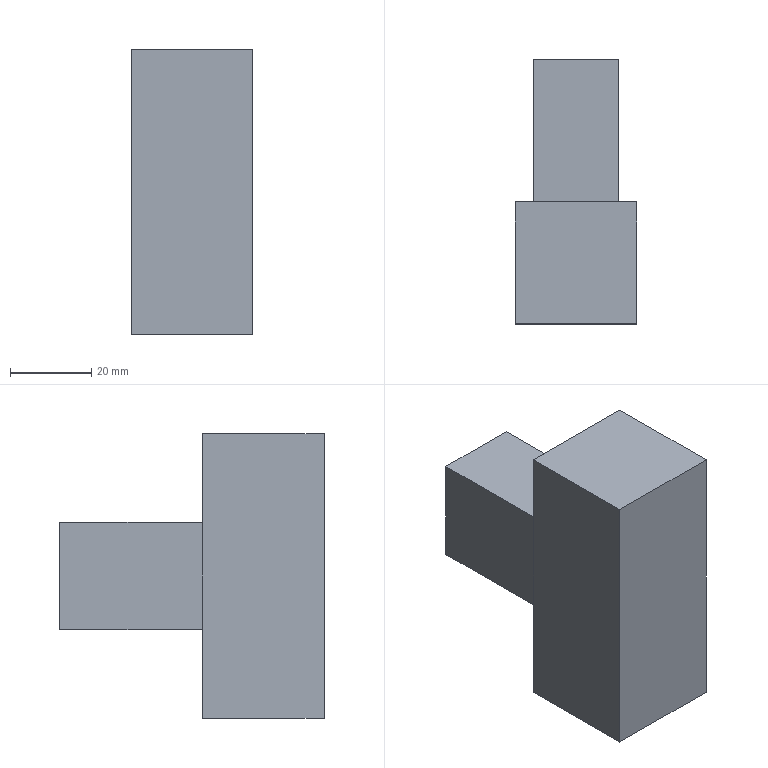Component | SolidWorks | HH54PIntermediateRelay-3 | 1 solid | 11 faces | box 30 x 65 x 70 mm | volume 82478 mm3 | plane 11
STEP:
#1=CARTESIAN_POINT('',(12.461,-0.7598,23.26));
#2=VERTEX_POINT('',#1);
#3=CARTESIAN_POINT('',(12.461,-0.7598,26.016));
#4=VERTEX_POINT('',#3);
#5=CARTESIAN_POINT('',(12.461,-0.7598,23.26));
#6=DIRECTION('',(0.,0.,1.));
#7=VECTOR('',#6,39.37);
#8=LINE('',#5,#7);
#9=EDGE_CURVE('',#2,#4,#8,.T.);
#10=ORIENTED_EDGE('',*,*,#9,.T.);
#11=CARTESIAN_POINT('',(13.643,-0.7598,26.016));
#12=VERTEX_POINT('',#11);
#13=CARTESIAN_POINT('',(12.461,-0.7598,26.016));
#14=DIRECTION('',(1.,0.,0.));
#15=VECTOR('',#14,39.37);
#16=LINE('',#13,#15);
#17=EDGE_CURVE('',#4,#12,#16,.T.);
#18=ORIENTED_EDGE('',*,*,#17,.T.);
#19=CARTESIAN_POINT('',(13.643,-0.7598,23.26));
#20=VERTEX_POINT('',#19);
#21=CARTESIAN_POINT('',(13.643,-0.7598,23.26));
#22=DIRECTION('',(-0.,-0.,-1.));
#23=VECTOR('',#22,39.37);
#24=LINE('',#21,#23);
#25=EDGE_CURVE('',#12,#20,#24,.T.);
#26=ORIENTED_EDGE('',*,*,#25,.T.);
#27=CARTESIAN_POINT('',(12.461,-0.7598,23.26));
#28=DIRECTION('',(-1.,0.,0.));
#29=VECTOR('',#28,39.37);
#30=LINE('',#27,#29);
#31=EDGE_CURVE('',#20,#2,#30,.T.);
#32=ORIENTED_EDGE('',*,*,#31,.T.);
#33=EDGE_LOOP('',(#10,#18,#26,#32));
#34=FACE_OUTER_BOUND('',#33,.T.);
#35=CARTESIAN_POINT('',(12.639,-0.7598,25.16));
#36=VERTEX_POINT('',#35);
#37=CARTESIAN_POINT('',(13.465,-0.7598,25.16));
#38=VERTEX_POINT('',#37);
#39=CARTESIAN_POINT('',(12.639,-0.7598,25.16));
#40=DIRECTION('',(1.,0.,0.));
#41=VECTOR('',#40,39.37);
#42=LINE('',#39,#41);
#43=EDGE_CURVE('',#36,#38,#42,.T.);
#44=ORIENTED_EDGE('',*,*,#43,.F.);
#45=CARTESIAN_POINT('',(12.639,-0.7598,24.116));
#46=VERTEX_POINT('',#45);
#47=CARTESIAN_POINT('',(12.639,-0.7598,24.116));
#48=DIRECTION('',(0.,0.,1.));
#49=VECTOR('',#48,39.37);
#50=LINE('',#47,#49);
#51=EDGE_CURVE('',#46,#36,#50,.T.);
#52=ORIENTED_EDGE('',*,*,#51,.F.);
#53=CARTESIAN_POINT('',(13.465,-0.7598,24.116));
#54=VERTEX_POINT('',#53);
#55=CARTESIAN_POINT('',(12.639,-0.7598,24.116));
#56=DIRECTION('',(-1.,0.,0.));
#57=VECTOR('',#56,39.37);
#58=LINE('',#55,#57);
#59=EDGE_CURVE('',#54,#46,#58,.T.);
#60=ORIENTED_EDGE('',*,*,#59,.F.);
#61=CARTESIAN_POINT('',(13.465,-0.7598,24.116));
#62=DIRECTION('',(-0.,-0.,-1.));
#63=VECTOR('',#62,39.37);
#64=LINE('',#61,#63);
#65=EDGE_CURVE('',#38,#54,#64,.T.);
#66=ORIENTED_EDGE('',*,*,#65,.F.);
#67=EDGE_LOOP('',(#44,#52,#60,#66));
#68=FACE_BOUND('',#67,.T.);
#69=CARTESIAN_POINT('',(13.267,-0.7598,24.309));
#70=DIRECTION('',(0.,1.,-0.));
#71=DIRECTION('',(1.,0.,0.));
#72=AXIS2_PLACEMENT_3D('',#69,#70,#71);
#73=PLANE('',#72);
#74=ADVANCED_FACE('',(#34,#68),#73,.T.);
#75=CARTESIAN_POINT('',(12.461,-1.941,23.26));
#76=VERTEX_POINT('',#75);
#77=CARTESIAN_POINT('',(12.461,-1.941,26.016));
#78=VERTEX_POINT('',#77);
#79=CARTESIAN_POINT('',(12.461,-1.941,23.26));
#80=DIRECTION('',(0.,0.,1.));
#81=VECTOR('',#80,39.37);
#82=LINE('',#79,#81);
#83=EDGE_CURVE('',#76,#78,#82,.T.);
#84=ORIENTED_EDGE('',*,*,#83,.T.);
#85=CARTESIAN_POINT('',(12.461,-0.7598,26.016));
#86=DIRECTION('',(0.,-1.,0.));
#87=VECTOR('',#86,39.37);
#88=LINE('',#85,#87);
#89=EDGE_CURVE('',#4,#78,#88,.T.);
#90=ORIENTED_EDGE('',*,*,#89,.F.);
#91=ORIENTED_EDGE('',*,*,#9,.F.);
#92=CARTESIAN_POINT('',(12.461,-0.7598,23.26));
#93=DIRECTION('',(0.,-1.,0.));
#94=VECTOR('',#93,39.37);
#95=LINE('',#92,#94);
#96=EDGE_CURVE('',#2,#76,#95,.T.);
#97=ORIENTED_EDGE('',*,*,#96,.T.);
#98=EDGE_LOOP('',(#84,#90,#91,#97));
#99=FACE_OUTER_BOUND('',#98,.T.);
#100=CARTESIAN_POINT('',(12.461,-0.7598,23.26));
#101=DIRECTION('',(1.,0.,0.));
#102=DIRECTION('',(0.,-1.,0.));
#103=AXIS2_PLACEMENT_3D('',#100,#101,#102);
#104=PLANE('',#103);
#105=ADVANCED_FACE('',(#99),#104,.F.);
#106=CARTESIAN_POINT('',(13.643,-1.941,26.016));
#107=VERTEX_POINT('',#106);
#108=CARTESIAN_POINT('',(12.461,-1.941,26.016));
#109=DIRECTION('',(1.,0.,0.));
#110=VECTOR('',#109,39.37);
#111=LINE('',#108,#110);
#112=EDGE_CURVE('',#78,#107,#111,.T.);
#113=ORIENTED_EDGE('',*,*,#112,.T.);
#114=CARTESIAN_POINT('',(13.643,-0.7598,26.016));
#115=DIRECTION('',(0.,-1.,0.));
#116=VECTOR('',#115,39.37);
#117=LINE('',#114,#116);
#118=EDGE_CURVE('',#12,#107,#117,.T.);
#119=ORIENTED_EDGE('',*,*,#118,.F.);
#120=ORIENTED_EDGE('',*,*,#17,.F.);
#121=ORIENTED_EDGE('',*,*,#89,.T.);
#122=EDGE_LOOP('',(#113,#119,#120,#121));
#123=FACE_OUTER_BOUND('',#122,.T.);
#124=CARTESIAN_POINT('',(12.461,-0.7598,26.016));
#125=DIRECTION('',(0.,-0.,-1.));
#126=DIRECTION('',(0.,1.,-0.));
#127=AXIS2_PLACEMENT_3D('',#124,#125,#126);
#128=PLANE('',#127);
#129=ADVANCED_FACE('',(#123),#128,.F.);
#130=CARTESIAN_POINT('',(13.643,-1.941,23.26));
#131=VERTEX_POINT('',#130);
#132=CARTESIAN_POINT('',(13.643,-1.941,23.26));
#133=DIRECTION('',(-0.,-0.,-1.));
#134=VECTOR('',#133,39.37);
#135=LINE('',#132,#134);
#136=EDGE_CURVE('',#107,#131,#135,.T.);
#137=ORIENTED_EDGE('',*,*,#136,.T.);
#138=CARTESIAN_POINT('',(13.643,-0.7598,23.26));
#139=DIRECTION('',(0.,-1.,0.));
#140=VECTOR('',#139,39.37);
#141=LINE('',#138,#140);
#142=EDGE_CURVE('',#20,#131,#141,.T.);
#143=ORIENTED_EDGE('',*,*,#142,.F.);
#144=ORIENTED_EDGE('',*,*,#25,.F.);
#145=ORIENTED_EDGE('',*,*,#118,.T.);
#146=EDGE_LOOP('',(#137,#143,#144,#145));
#147=FACE_OUTER_BOUND('',#146,.T.);
#148=CARTESIAN_POINT('',(13.643,-0.7598,23.26));
#149=DIRECTION('',(-1.,0.,0.));
#150=DIRECTION('',(0.,0.,1.));
#151=AXIS2_PLACEMENT_3D('',#148,#149,#150);
#152=PLANE('',#151);
#153=ADVANCED_FACE('',(#147),#152,.F.);
#154=CARTESIAN_POINT('',(12.461,-1.941,23.26));
#155=DIRECTION('',(-1.,0.,0.));
#156=VECTOR('',#155,39.37);
#157=LINE('',#154,#156);
#158=EDGE_CURVE('',#131,#76,#157,.T.);
#159=ORIENTED_EDGE('',*,*,#158,.T.);
#160=ORIENTED_EDGE('',*,*,#96,.F.);
#161=ORIENTED_EDGE('',*,*,#31,.F.);
#162=ORIENTED_EDGE('',*,*,#142,.T.);
#163=EDGE_LOOP('',(#159,#160,#161,#162));
#164=FACE_OUTER_BOUND('',#163,.T.);
#165=CARTESIAN_POINT('',(12.461,-0.7598,23.26));
#166=DIRECTION('',(0.,0.,1.));
#167=DIRECTION('',(0.,-1.,0.));
#168=AXIS2_PLACEMENT_3D('',#165,#166,#167);
#169=PLANE('',#168);
#170=ADVANCED_FACE('',(#164),#169,.F.);
#171=ORIENTED_EDGE('',*,*,#83,.F.);
#172=ORIENTED_EDGE('',*,*,#158,.F.);
#173=ORIENTED_EDGE('',*,*,#136,.F.);
#174=ORIENTED_EDGE('',*,*,#112,.F.);
#175=EDGE_LOOP('',(#171,#172,#173,#174));
#176=FACE_OUTER_BOUND('',#175,.T.);
#177=CARTESIAN_POINT('',(13.267,-1.941,24.309));
#178=DIRECTION('',(0.,1.,-0.));
#179=DIRECTION('',(1.,0.,0.));
#180=AXIS2_PLACEMENT_3D('',#177,#178,#179);
#181=PLANE('',#180);
#182=ADVANCED_FACE('',(#176),#181,.F.);
#183=ORIENTED_EDGE('',*,*,#51,.T.);
#184=CARTESIAN_POINT('',(12.639,0.6182,25.16));
#185=VERTEX_POINT('',#184);
#186=CARTESIAN_POINT('',(12.639,0.6182,25.16));
#187=DIRECTION('',(0.,-1.,0.));
#188=VECTOR('',#187,39.37);
#189=LINE('',#186,#188);
#190=EDGE_CURVE('',#185,#36,#189,.T.);
#191=ORIENTED_EDGE('',*,*,#190,.F.);
#192=CARTESIAN_POINT('',(12.639,0.6182,24.116));
#193=VERTEX_POINT('',#192);
#194=CARTESIAN_POINT('',(12.639,0.6182,24.116));
#195=DIRECTION('',(0.,0.,1.));
#196=VECTOR('',#195,39.37);
#197=LINE('',#194,#196);
#198=EDGE_CURVE('',#193,#185,#197,.T.);
#199=ORIENTED_EDGE('',*,*,#198,.F.);
#200=CARTESIAN_POINT('',(12.639,0.6182,24.116));
#201=DIRECTION('',(0.,-1.,0.));
#202=VECTOR('',#201,39.37);
#203=LINE('',#200,#202);
#204=EDGE_CURVE('',#193,#46,#203,.T.);
#205=ORIENTED_EDGE('',*,*,#204,.T.);
#206=EDGE_LOOP('',(#183,#191,#199,#205));
#207=FACE_OUTER_BOUND('',#206,.T.);
#208=CARTESIAN_POINT('',(12.639,0.6182,24.116));
#209=DIRECTION('',(1.,-0.,-0.));
#210=DIRECTION('',(-0.,-0.,-1.));
#211=AXIS2_PLACEMENT_3D('',#208,#209,#210);
#212=PLANE('',#211);
#213=ADVANCED_FACE('',(#207),#212,.F.);
#214=ORIENTED_EDGE('',*,*,#43,.T.);
#215=CARTESIAN_POINT('',(13.465,0.6182,25.16));
#216=VERTEX_POINT('',#215);
#217=CARTESIAN_POINT('',(13.465,0.6182,25.16));
#218=DIRECTION('',(0.,-1.,0.));
#219=VECTOR('',#218,39.37);
#220=LINE('',#217,#219);
#221=EDGE_CURVE('',#216,#38,#220,.T.);
#222=ORIENTED_EDGE('',*,*,#221,.F.);
#223=CARTESIAN_POINT('',(12.639,0.6182,25.16));
#224=DIRECTION('',(1.,0.,0.));
#225=VECTOR('',#224,39.37);
#226=LINE('',#223,#225);
#227=EDGE_CURVE('',#185,#216,#226,.T.);
#228=ORIENTED_EDGE('',*,*,#227,.F.);
#229=ORIENTED_EDGE('',*,*,#190,.T.);
#230=EDGE_LOOP('',(#214,#222,#228,#229));
#231=FACE_OUTER_BOUND('',#230,.T.);
#232=CARTESIAN_POINT('',(12.639,0.6182,25.16));
#233=DIRECTION('',(0.,-0.,-1.));
#234=DIRECTION('',(-1.,-0.,-0.));
#235=AXIS2_PLACEMENT_3D('',#232,#233,#234);
#236=PLANE('',#235);
#237=ADVANCED_FACE('',(#231),#236,.F.);
#238=ORIENTED_EDGE('',*,*,#65,.T.);
#239=CARTESIAN_POINT('',(13.465,0.6182,24.116));
#240=VERTEX_POINT('',#239);
#241=CARTESIAN_POINT('',(13.465,0.6182,24.116));
#242=DIRECTION('',(0.,-1.,0.));
#243=VECTOR('',#242,39.37);
#244=LINE('',#241,#243);
#245=EDGE_CURVE('',#240,#54,#244,.T.);
#246=ORIENTED_EDGE('',*,*,#245,.F.);
#247=CARTESIAN_POINT('',(13.465,0.6182,24.116));
#248=DIRECTION('',(-0.,-0.,-1.));
#249=VECTOR('',#248,39.37);
#250=LINE('',#247,#249);
#251=EDGE_CURVE('',#216,#240,#250,.T.);
#252=ORIENTED_EDGE('',*,*,#251,.F.);
#253=ORIENTED_EDGE('',*,*,#221,.T.);
#254=EDGE_LOOP('',(#238,#246,#252,#253));
#255=FACE_OUTER_BOUND('',#254,.T.);
#256=CARTESIAN_POINT('',(13.465,0.6182,24.116));
#257=DIRECTION('',(-1.,0.,0.));
#258=DIRECTION('',(0.,0.,1.));
#259=AXIS2_PLACEMENT_3D('',#256,#257,#258);
#260=PLANE('',#259);
#261=ADVANCED_FACE('',(#255),#260,.F.);
#262=ORIENTED_EDGE('',*,*,#59,.T.);
#263=ORIENTED_EDGE('',*,*,#204,.F.);
#264=CARTESIAN_POINT('',(12.639,0.6182,24.116));
#265=DIRECTION('',(-1.,0.,0.));
#266=VECTOR('',#265,39.37);
#267=LINE('',#264,#266);
#268=EDGE_CURVE('',#240,#193,#267,.T.);
#269=ORIENTED_EDGE('',*,*,#268,.F.);
#270=ORIENTED_EDGE('',*,*,#245,.T.);
#271=EDGE_LOOP('',(#262,#263,#269,#270));
#272=FACE_OUTER_BOUND('',#271,.T.);
#273=CARTESIAN_POINT('',(12.639,0.6182,24.116));
#274=DIRECTION('',(0.,0.,1.));
#275=DIRECTION('',(0.,-1.,0.));
#276=AXIS2_PLACEMENT_3D('',#273,#274,#275);
#277=PLANE('',#276);
#278=ADVANCED_FACE('',(#272),#277,.F.);
#279=ORIENTED_EDGE('',*,*,#198,.T.);
#280=ORIENTED_EDGE('',*,*,#227,.T.);
#281=ORIENTED_EDGE('',*,*,#251,.T.);
#282=ORIENTED_EDGE('',*,*,#268,.T.);
#283=EDGE_LOOP('',(#279,#280,#281,#282));
#284=FACE_OUTER_BOUND('',#283,.T.);
#285=CARTESIAN_POINT('',(13.267,0.6182,24.309));
#286=DIRECTION('',(0.,1.,-0.));
#287=DIRECTION('',(1.,0.,0.));
#288=AXIS2_PLACEMENT_3D('',#285,#286,#287);
#289=PLANE('',#288);
#290=ADVANCED_FACE('',(#284),#289,.T.);
#291=CLOSED_SHELL('',(#74,#105,#129,#153,#170,#182,#213,#237,#261,#278,#290));
#292=MANIFOLD_SOLID_BREP('',#291);
#293=CARTESIAN_POINT('',(0.,0.,0.));
#294=DIRECTION('',(0.,0.,1.));
#295=DIRECTION('',(1.,0.,0.));
#296=AXIS2_PLACEMENT_3D('',#293,#294,#295);
#297=(LENGTH_UNIT()NAMED_UNIT(*)SI_UNIT($,.METRE.));
#298=LENGTH_MEASURE_WITH_UNIT(LENGTH_MEASURE(0.0254),#297);
#299=DIMENSIONAL_EXPONENTS(1.,0.,0.,0.,0.,0.,0.);
#300=(CONVERSION_BASED_UNIT('',#298)LENGTH_UNIT()NAMED_UNIT(#299));
#301=UNCERTAINTY_MEASURE_WITH_UNIT(LENGTH_MEASURE(0.00001),#300,'','');
#302=(NAMED_UNIT(*)PLANE_ANGLE_UNIT()SI_UNIT($,.RADIAN.));
#303=(NAMED_UNIT(*)SI_UNIT($,.STERADIAN.)SOLID_ANGLE_UNIT());
#304=(GEOMETRIC_REPRESENTATION_CONTEXT(3)GLOBAL_UNCERTAINTY_ASSIGNED_CONTEXT((#301))GLOBAL_UNIT_ASSIGNED_CONTEXT((#300,#302,#303))REPRESENTATION_CONTEXT('',''));
#305=ADVANCED_BREP_SHAPE_REPRESENTATION('',(#292,#296),#304);
#306=COLOUR_RGB('',0.7922,0.8196,0.9333);
#307=FILL_AREA_STYLE_COLOUR('',#306);
#308=FILL_AREA_STYLE('',(#307));
#309=SURFACE_STYLE_FILL_AREA(#308);
#310=SURFACE_SIDE_STYLE('',(#309));
#311=SURFACE_STYLE_USAGE(.BOTH.,#310);
#312=PRESENTATION_STYLE_ASSIGNMENT((#311));
#313=STYLED_ITEM('',(#312),#292);
#314=PRESENTATION_LAYER_ASSIGNMENT('','',(#313));
#315=(LENGTH_UNIT()NAMED_UNIT(*)SI_UNIT($,.METRE.));
#316=LENGTH_MEASURE_WITH_UNIT(LENGTH_MEASURE(0.0254),#315);
#317=DIMENSIONAL_EXPONENTS(1.,0.,0.,0.,0.,0.,0.);
#318=(CONVERSION_BASED_UNIT('',#316)LENGTH_UNIT()NAMED_UNIT(#317));
#319=UNCERTAINTY_MEASURE_WITH_UNIT(LENGTH_MEASURE(0.00001),#318,'','');
#320=(NAMED_UNIT(*)PLANE_ANGLE_UNIT()SI_UNIT($,.RADIAN.));
#321=(NAMED_UNIT(*)SI_UNIT($,.STERADIAN.)SOLID_ANGLE_UNIT());
#322=(GEOMETRIC_REPRESENTATION_CONTEXT(3)GLOBAL_UNCERTAINTY_ASSIGNED_CONTEXT((#319))GLOBAL_UNIT_ASSIGNED_CONTEXT((#318,#320,#321))REPRESENTATION_CONTEXT('',''));
#323=MECHANICAL_DESIGN_GEOMETRIC_PRESENTATION_REPRESENTATION('',(#313),#322);